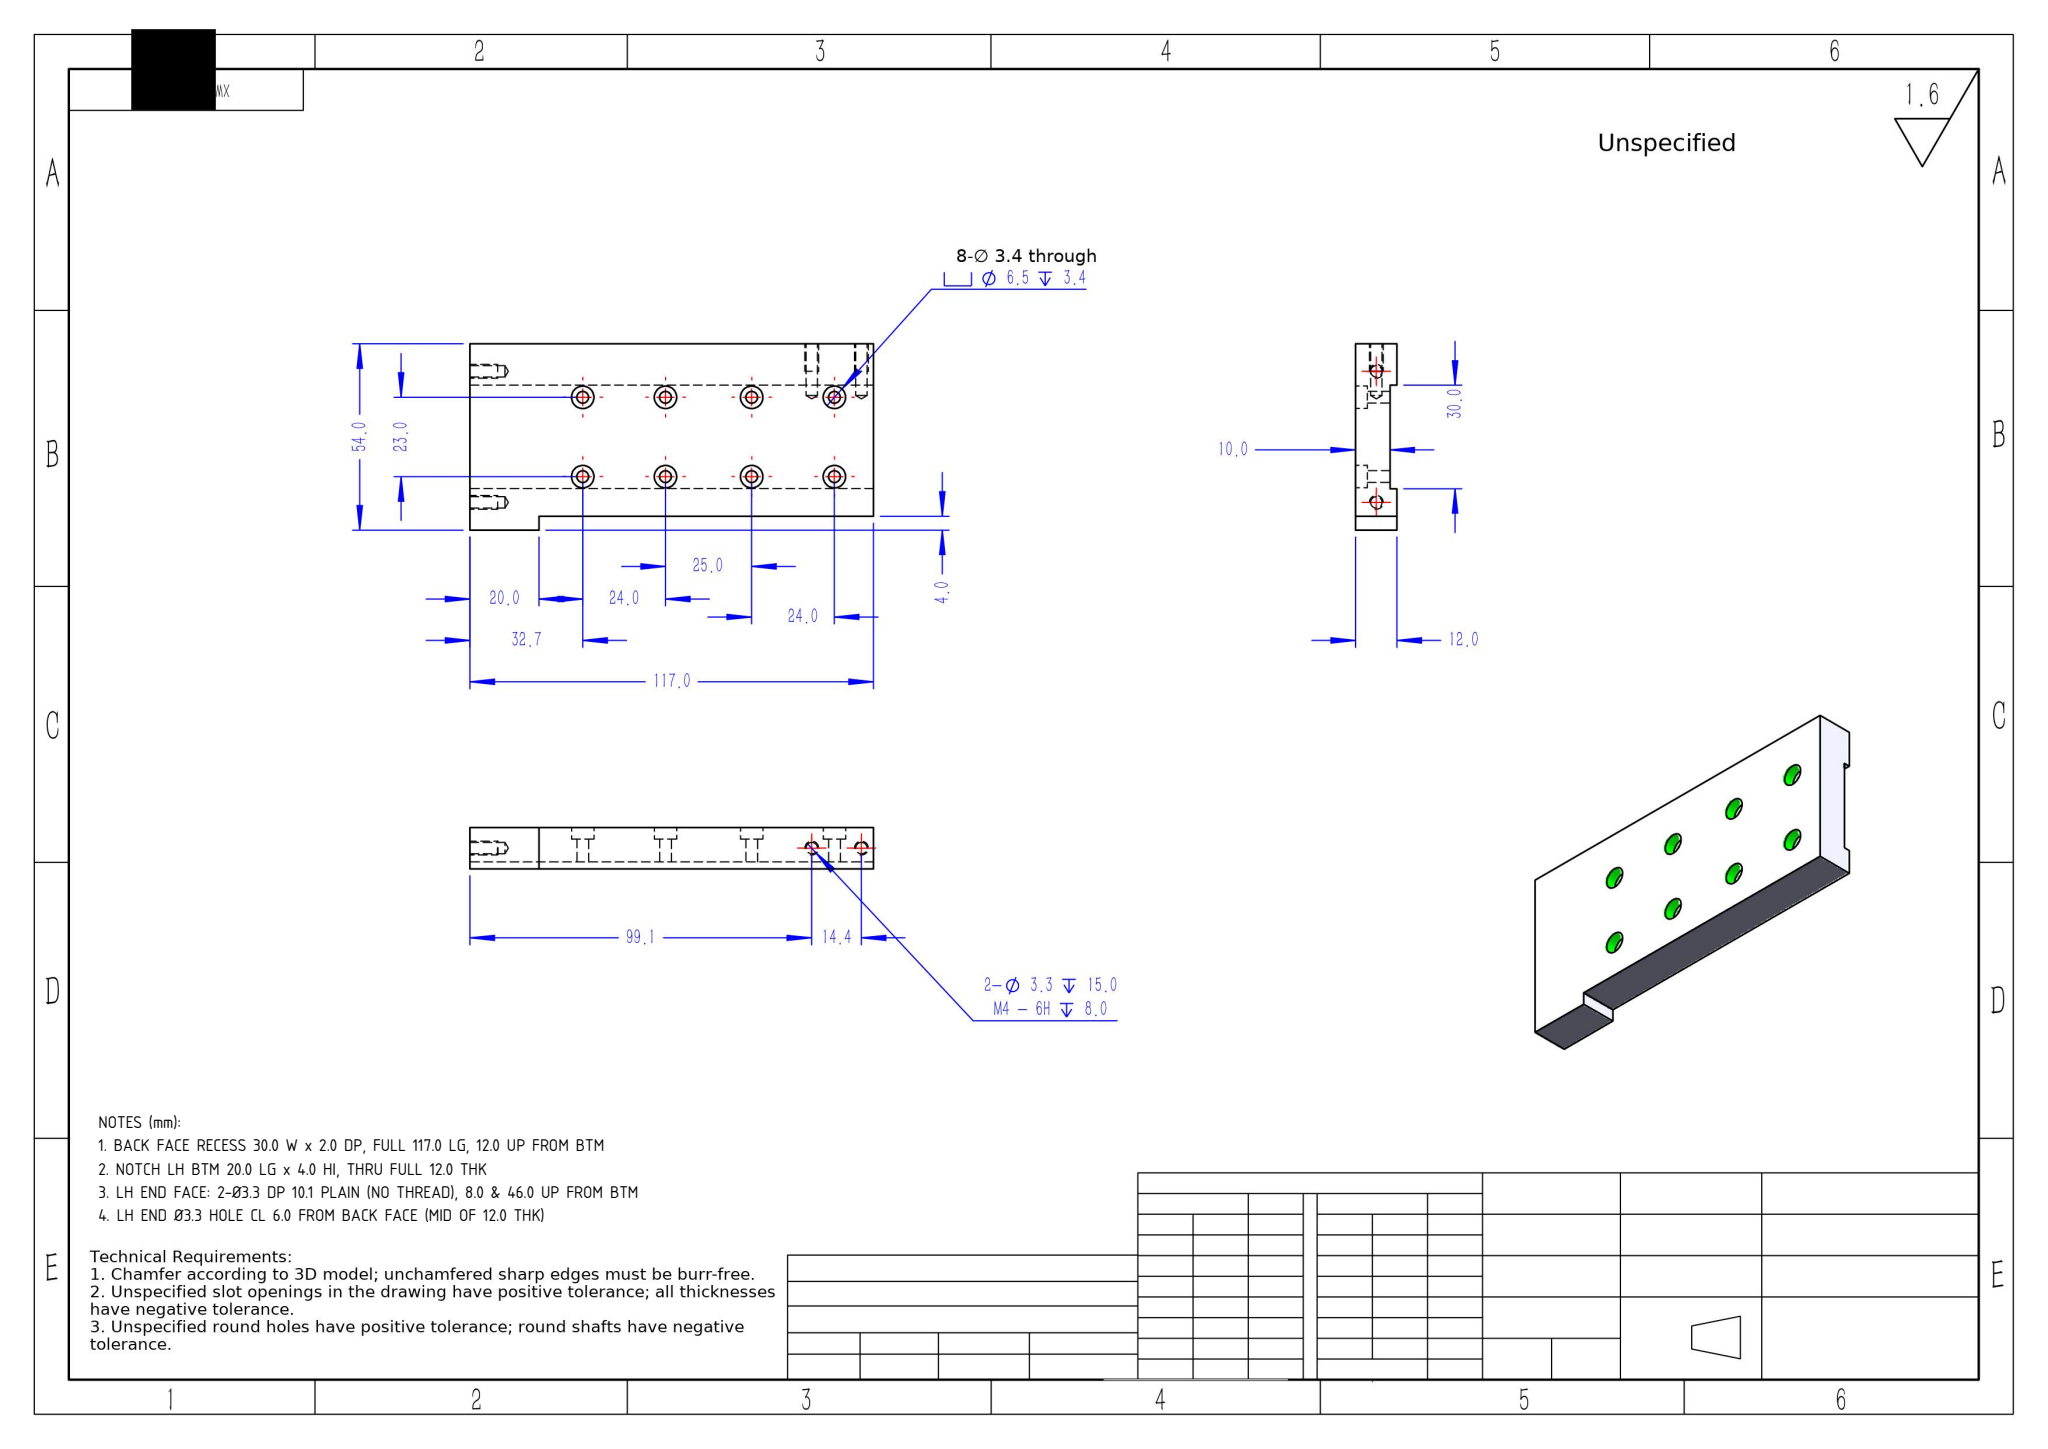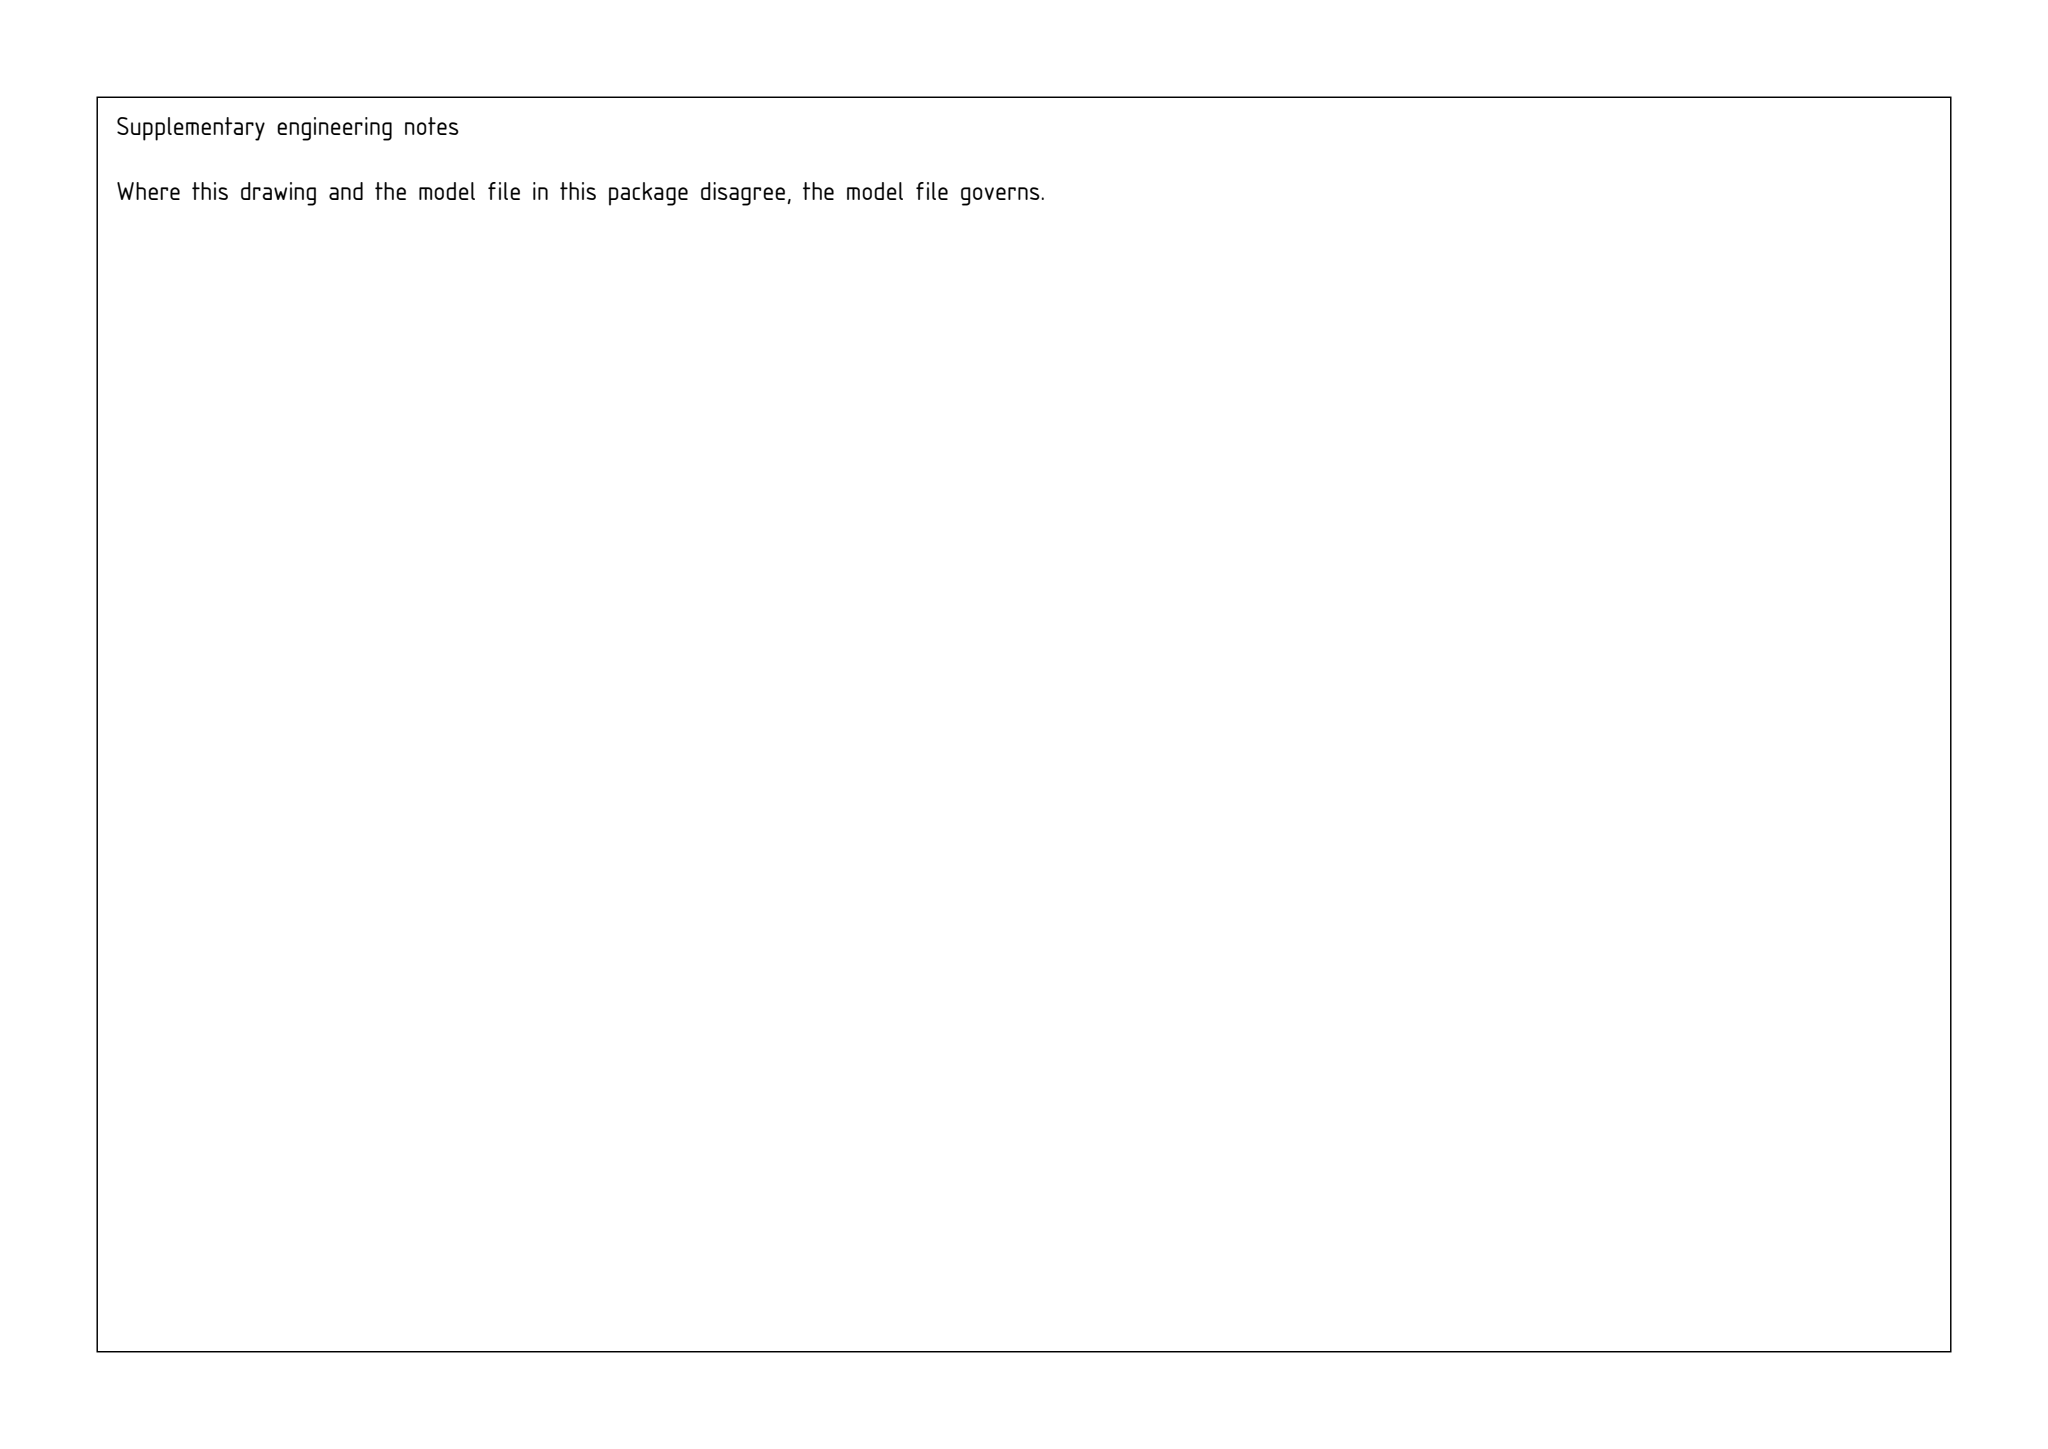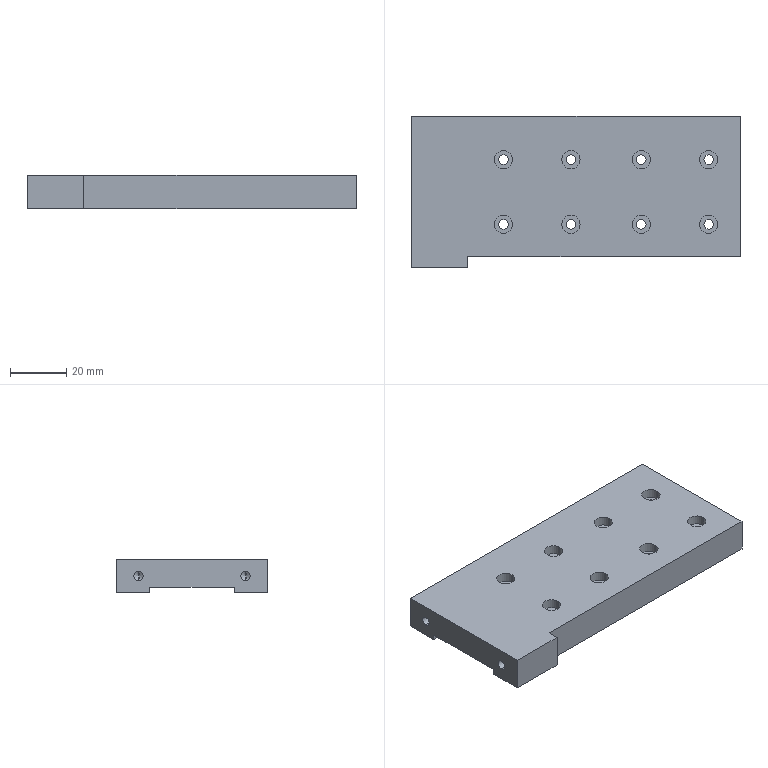Part | SolidWorks | mm | 1 solid | 68 faces | box 117 x 54 x 12 mm | volume 62317 mm3 | cylinder 40 | plane 20 | cone 8 | commonest cylinder face diameters 6.5 x16 3.4 x16 3.3 x8
Drawing notes:
BACK FACE RECESS 30.0 W x 2.0 DP, FULL 117.0 LG, 12.0 UP FROM BTM | from the solid: y planes 12.0 & 42.0 (30 apart), z plane 2.0 below back face z=0, runs x=0-117
NOTCH LH BTM 20.0 LG x 4.0 HI, THRU FULL 12.0 THK | from the solid: x plane 20.0 and y plane 4.0 at min corner; y=0 face only x=20-117; full z 0-12
LH END FACE: 2-Ø3.3 DP 10.1 PLAIN (NO THREAD), 8.0 & 46.0 UP FROM BTM | from the solid: cyl Ø3.3 axis x, len 10.1, at y=8.0 & 46.0; 118 deg drill point cones ref dia 3.3
LH END Ø3.3 HOLE CL 6.0 FROM BACK FACE (MID OF 12.0 THK) | from the solid: cyl Ø3.3 axis x at z=6.0; bbox Z=12.0
build123d program:
from build123d import *

# Parameters (mm, degrees)
SKETCH1_W                                       = 117
SKETCH1_H                                       = 54
BOSS_EXTRUDE1_DEPTH                             = 6
SKETCH2_W                                       = 117
SKETCH2_H                                       = 30
CUT_EXTRUDE1_DEPTH                              = 2
SKETCH4_W                                       = 97
SKETCH4_H                                       = 12
CUT_EXTRUDE3_DEPTH                              = 4
M3_HEX_SOCKET_HEAD_CAP_SCREW_CBORE1_D           = 3.4
M3_HEX_SOCKET_HEAD_CAP_SCREW_CBORE1_DEPTH       = 12
M3_HEX_SOCKET_HEAD_CAP_SCREW_CBORE1_CBORE_D     = 6.5
M3_HEX_SOCKET_HEAD_CAP_SCREW_CBORE1_CBORE_DEPTH = 3.4
M4_TAPPED_HOLE2_D                               = 3.3
M4_TAPPED_HOLE2_DEPTH                           = 15
M4_TAPPED_HOLE2_TIP                             = 0.9914


with BuildPart() as part:
    # Sketch1 → Boss-Extrude1 (new, symmetric)
    with BuildSketch(Plane.XY):
        Rectangle(SKETCH1_W, SKETCH1_H)
    extrude(amount=BOSS_EXTRUDE1_DEPTH, both=True)

    # Sketch2 → Cut-Extrude1 (cut)
    with BuildSketch(Plane(origin=(0, 0, -6), x_dir=(-1, 0, 0), z_dir=(0, 0, -1))):
        Rectangle(SKETCH2_W, SKETCH2_H)
    extrude(amount=-CUT_EXTRUDE1_DEPTH, mode=Mode.SUBTRACT)

    # Sketch4 → Cut-Extrude3 (cut)
    with BuildSketch(Plane.XZ.offset(27)):
        with Locations((10, 0)):
            Rectangle(SKETCH4_W, SKETCH4_H)
    extrude(amount=-CUT_EXTRUDE3_DEPTH, mode=Mode.SUBTRACT)

    # M3 Hex Socket Head Cap Screw CBORE1
    with Locations(Plane.XY.offset(6)):
        with Locations((-1.8, -11.5), (-25.8, -11.5), (-25.8, 11.5), (-1.8, 11.5), (47.2, -11.5), (23.2, -11.5), (23.2, 11.5), (47.2, 11.5)):
            CounterBoreHole(M3_HEX_SOCKET_HEAD_CAP_SCREW_CBORE1_D / 2, M3_HEX_SOCKET_HEAD_CAP_SCREW_CBORE1_CBORE_D / 2, M3_HEX_SOCKET_HEAD_CAP_SCREW_CBORE1_CBORE_DEPTH, depth=M3_HEX_SOCKET_HEAD_CAP_SCREW_CBORE1_DEPTH)

    # Sketch10 → M4 Tapped Hole1 (revolve, cut)
    with BuildSketch(Plane(origin=(-58.5, -19, 0), x_dir=(0, 0, 1), z_dir=(0, 1, 0))):
        Polygon((0, 0), (0, 11.091), (1.65, 10.1), (1.65, 0), align=None)
    m4_tapped_hole1 = revolve(axis=Axis((-64.85, -19, 0), (1, 0, 0)), mode=Mode.SUBTRACT)

    # Mirror1: M4 Tapped Hole1 across plane
    add(m4_tapped_hole1.mirror(Plane.ZX), mode=Mode.SUBTRACT)

    # M4 Tapped Hole2
    with Locations(Plane(origin=(0, 27, 0), x_dir=(1, 0, 0), z_dir=(0, 1, 0))):
        with Locations((55, 0), (40.6, 0)):
            Hole(M4_TAPPED_HOLE2_D / 2, depth=M4_TAPPED_HOLE2_DEPTH)
            with Locations((0, 0, -(M4_TAPPED_HOLE2_DEPTH + M4_TAPPED_HOLE2_TIP / 2))):  # 118° drill point
                Cone(0, M4_TAPPED_HOLE2_D / 2, M4_TAPPED_HOLE2_TIP, mode=Mode.SUBTRACT)


solid = part.part